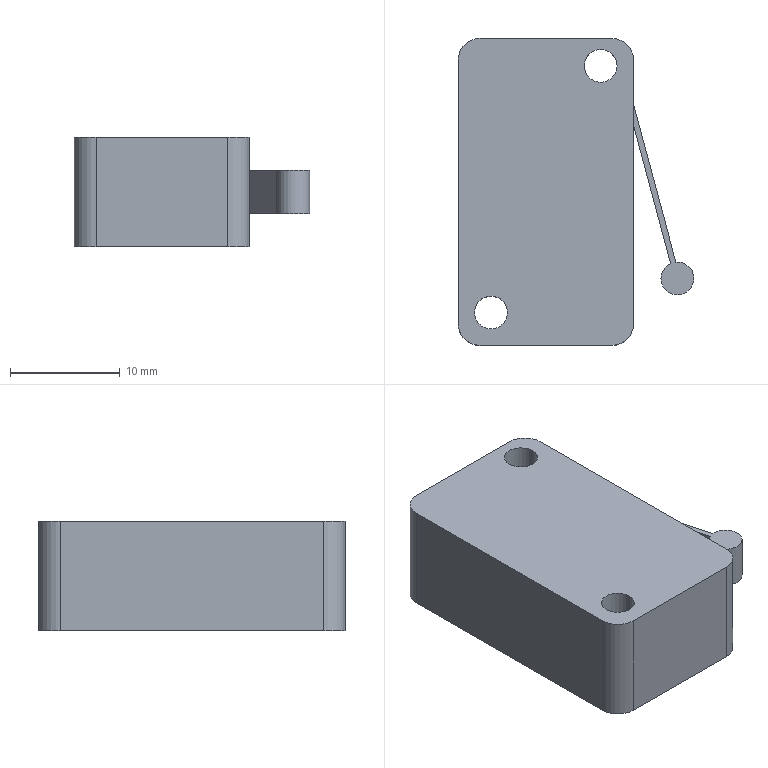Component | SolidWorks | MicroSwitch-1 | 2 solids | 22 faces | box 21.5 x 28 x 10 mm | volume 4360 mm3 | cylinder 11 | plane 11 | commonest cylinder face diameters 3 x7 4 x4
build123d program:
from build123d import *

# Parameters (mm, degrees)
SKETCH1_W      = 28
SKETCH1_H      = 16
EXTRUDE1_DEPTH = 5
SKETCH2_R      = 1.5
EXTRUDE2_DEPTH = 34.764
EXTRUDE3_DEPTH = 2
FILLET1_R      = 2


with BuildPart() as part:
    # Sketch1 → Extrude1 (new, symmetric)
    with BuildSketch(Plane(origin=(0, 0, 0), x_dir=(1, 0, 0), z_dir=(0, 1, 0))):
        with Locations((14, 8)):
            Rectangle(SKETCH1_W, SKETCH1_H)
    extrude(amount=EXTRUDE1_DEPTH, both=True)

    # Sketch2 → Extrude2 (cut, through all)
    with BuildSketch(Plane(origin=(0, 5, 0), x_dir=(1, 0, 0), z_dir=(0, 1, 0))):
        with Locations(Location((25.5, 13, 0), (0, 0, 270))):
            Circle(SKETCH2_R)
        with Locations(Location((3, 3, 0), (0, 0, 270))):
            Circle(SKETCH2_R)
    extrude(amount=-EXTRUDE2_DEPTH, mode=Mode.SUBTRACT)

    # Fillet1
    fillet1_edges = [part.edges().sort_by_distance(p)[0] for p in [
        (0, 0, -16),
        (28, 0, -16),
        (28, 0, 0),
        (0, 0, 0),
    ]]
    fillet(fillet1_edges, radius=FILLET1_R)


with BuildPart() as body_2:
    # Sketch3 → Extrude3 (new, symmetric)
    with BuildSketch(Plane(origin=(0, 0, 0), x_dir=(1, 0, 0), z_dir=(0, 1, 0))):
        with BuildLine():
            Line((7.599, 19.859), (22, 16))
            Line((22, 16), (20.068, 16))
            Line((20.068, 16), (7.47, 19.376))
            ThreePointArc((7.47, 19.376), (4.657, 20.388), (7.599, 19.859))
        make_face()
    extrude(amount=EXTRUDE3_DEPTH, both=True)


solid = Compound([part.part, body_2.part])

# Placed as in the assembly
solid = solid.moved(Location((-20.734, 63.799, 41), (-90, -90, 0)))
STEP:
#1=COLOUR_RGB('',0.7922,0.8196,0.9333);
#2=FILL_AREA_STYLE_COLOUR('',#1);
#3=FILL_AREA_STYLE('',(#2));
#4=SURFACE_STYLE_FILL_AREA(#3);
#5=SURFACE_SIDE_STYLE('',(#4));
#6=SURFACE_STYLE_USAGE(.BOTH.,#5);
#7=PRESENTATION_STYLE_ASSIGNMENT((#6));
#8=CARTESIAN_POINT('',(-0.6391,2.63,1.811));
#9=VERTEX_POINT('',#8);
#10=CARTESIAN_POINT('',(-0.7572,2.63,1.811));
#11=VERTEX_POINT('',#10);
#12=CARTESIAN_POINT('',(-0.6982,2.63,1.811));
#13=DIRECTION('',(-0.,0.,-1.));
#14=DIRECTION('',(-1.,0.,0.));
#15=AXIS2_PLACEMENT_3D('',#12,#13,#14);
#16=CIRCLE('',#15,0.05906);
#17=EDGE_CURVE('',#9,#11,#16,.T.);
#18=ORIENTED_EDGE('',*,*,#17,.F.);
#19=CARTESIAN_POINT('',(-0.6391,2.63,1.417));
#20=VERTEX_POINT('',#19);
#21=CARTESIAN_POINT('',(-0.6391,2.63,1.811));
#22=DIRECTION('',(-0.,0.,-1.));
#23=VECTOR('',#22,39.37);
#24=LINE('',#21,#23);
#25=EDGE_CURVE('',#9,#20,#24,.T.);
#26=ORIENTED_EDGE('',*,*,#25,.T.);
#27=CARTESIAN_POINT('',(-0.7572,2.63,1.417));
#28=VERTEX_POINT('',#27);
#29=CARTESIAN_POINT('',(-0.6982,2.63,1.417));
#30=DIRECTION('',(-0.,0.,-1.));
#31=DIRECTION('',(-1.,0.,0.));
#32=AXIS2_PLACEMENT_3D('',#29,#30,#31);
#33=CIRCLE('',#32,0.05906);
#34=EDGE_CURVE('',#20,#28,#33,.T.);
#35=ORIENTED_EDGE('',*,*,#34,.T.);
#36=CARTESIAN_POINT('',(-0.7572,2.63,1.811));
#37=DIRECTION('',(-0.,0.,-1.));
#38=VECTOR('',#37,39.37);
#39=LINE('',#36,#38);
#40=EDGE_CURVE('',#11,#28,#39,.T.);
#41=ORIENTED_EDGE('',*,*,#40,.F.);
#42=EDGE_LOOP('',(#18,#26,#35,#41));
#43=FACE_OUTER_BOUND('',#42,.T.);
#44=CARTESIAN_POINT('',(-0.6982,2.63,1.811));
#45=DIRECTION('',(-0.,0.,-1.));
#46=DIRECTION('',(-1.,0.,0.));
#47=AXIS2_PLACEMENT_3D('',#44,#45,#46);
#48=CYLINDRICAL_SURFACE('',#47,0.05906);
#49=ADVANCED_FACE('',(#43),#48,.F.);
#50=CARTESIAN_POINT('',(-0.2454,3.516,1.811));
#51=VERTEX_POINT('',#50);
#52=CARTESIAN_POINT('',(-0.3635,3.516,1.811));
#53=VERTEX_POINT('',#52);
#54=CARTESIAN_POINT('',(-0.3045,3.516,1.811));
#55=DIRECTION('',(-0.,0.,-1.));
#56=DIRECTION('',(-1.,0.,0.));
#57=AXIS2_PLACEMENT_3D('',#54,#55,#56);
#58=CIRCLE('',#57,0.05906);
#59=EDGE_CURVE('',#51,#53,#58,.T.);
#60=ORIENTED_EDGE('',*,*,#59,.F.);
#61=CARTESIAN_POINT('',(-0.2454,3.516,1.417));
#62=VERTEX_POINT('',#61);
#63=CARTESIAN_POINT('',(-0.2454,3.516,1.811));
#64=DIRECTION('',(-0.,0.,-1.));
#65=VECTOR('',#64,39.37);
#66=LINE('',#63,#65);
#67=EDGE_CURVE('',#51,#62,#66,.T.);
#68=ORIENTED_EDGE('',*,*,#67,.T.);
#69=CARTESIAN_POINT('',(-0.3635,3.516,1.417));
#70=VERTEX_POINT('',#69);
#71=CARTESIAN_POINT('',(-0.3045,3.516,1.417));
#72=DIRECTION('',(-0.,0.,-1.));
#73=DIRECTION('',(-1.,0.,0.));
#74=AXIS2_PLACEMENT_3D('',#71,#72,#73);
#75=CIRCLE('',#74,0.05906);
#76=EDGE_CURVE('',#62,#70,#75,.T.);
#77=ORIENTED_EDGE('',*,*,#76,.T.);
#78=CARTESIAN_POINT('',(-0.3635,3.516,1.811));
#79=DIRECTION('',(-0.,0.,-1.));
#80=VECTOR('',#79,39.37);
#81=LINE('',#78,#80);
#82=EDGE_CURVE('',#53,#70,#81,.T.);
#83=ORIENTED_EDGE('',*,*,#82,.F.);
#84=EDGE_LOOP('',(#60,#68,#77,#83));
#85=FACE_OUTER_BOUND('',#84,.T.);
#86=CARTESIAN_POINT('',(-0.3045,3.516,1.811));
#87=DIRECTION('',(-0.,0.,-1.));
#88=DIRECTION('',(-1.,0.,0.));
#89=AXIS2_PLACEMENT_3D('',#86,#87,#88);
#90=CYLINDRICAL_SURFACE('',#89,0.05906);
#91=ADVANCED_FACE('',(#85),#90,.F.);
#92=CARTESIAN_POINT('',(-0.2651,2.512,1.811));
#93=VERTEX_POINT('',#92);
#94=CARTESIAN_POINT('',(-0.7375,2.512,1.811));
#95=VERTEX_POINT('',#94);
#96=CARTESIAN_POINT('',(-0.8163,2.512,1.811));
#97=DIRECTION('',(-1.,-0.,0.));
#98=VECTOR('',#97,39.37);
#99=LINE('',#96,#98);
#100=EDGE_CURVE('',#93,#95,#99,.T.);
#101=ORIENTED_EDGE('',*,*,#100,.T.);
#102=CARTESIAN_POINT('',(-0.7375,2.512,1.417));
#103=VERTEX_POINT('',#102);
#104=CARTESIAN_POINT('',(-0.7375,2.512,1.417));
#105=DIRECTION('',(-0.,0.,-1.));
#106=VECTOR('',#105,39.37);
#107=LINE('',#104,#106);
#108=EDGE_CURVE('',#95,#103,#107,.T.);
#109=ORIENTED_EDGE('',*,*,#108,.T.);
#110=CARTESIAN_POINT('',(-0.2651,2.512,1.417));
#111=VERTEX_POINT('',#110);
#112=CARTESIAN_POINT('',(-0.8163,2.512,1.417));
#113=DIRECTION('',(-1.,-0.,0.));
#114=VECTOR('',#113,39.37);
#115=LINE('',#112,#114);
#116=EDGE_CURVE('',#111,#103,#115,.T.);
#117=ORIENTED_EDGE('',*,*,#116,.F.);
#118=CARTESIAN_POINT('',(-0.2651,2.512,1.417));
#119=DIRECTION('',(0.,-0.,1.));
#120=VECTOR('',#119,39.37);
#121=LINE('',#118,#120);
#122=EDGE_CURVE('',#111,#93,#121,.T.);
#123=ORIENTED_EDGE('',*,*,#122,.T.);
#124=EDGE_LOOP('',(#101,#109,#117,#123));
#125=FACE_OUTER_BOUND('',#124,.T.);
#126=CARTESIAN_POINT('',(-0.8163,2.512,1.417));
#127=DIRECTION('',(-0.,1.,0.));
#128=DIRECTION('',(1.,0.,-0.));
#129=AXIS2_PLACEMENT_3D('',#126,#127,#128);
#130=PLANE('',#129);
#131=ADVANCED_FACE('',(#125),#130,.F.);
#132=CARTESIAN_POINT('',(-0.8163,2.591,1.417));
#133=VERTEX_POINT('',#132);
#134=CARTESIAN_POINT('',(-0.8163,3.535,1.417));
#135=VERTEX_POINT('',#134);
#136=CARTESIAN_POINT('',(-0.8163,2.512,1.417));
#137=DIRECTION('',(-0.,1.,0.));
#138=VECTOR('',#137,39.37);
#139=LINE('',#136,#138);
#140=EDGE_CURVE('',#133,#135,#139,.T.);
#141=ORIENTED_EDGE('',*,*,#140,.F.);
#142=CARTESIAN_POINT('',(-0.8163,2.591,1.811));
#143=VERTEX_POINT('',#142);
#144=CARTESIAN_POINT('',(-0.8163,2.591,1.417));
#145=DIRECTION('',(0.,-0.,1.));
#146=VECTOR('',#145,39.37);
#147=LINE('',#144,#146);
#148=EDGE_CURVE('',#133,#143,#147,.T.);
#149=ORIENTED_EDGE('',*,*,#148,.T.);
#150=CARTESIAN_POINT('',(-0.8163,3.535,1.811));
#151=VERTEX_POINT('',#150);
#152=CARTESIAN_POINT('',(-0.8163,2.512,1.811));
#153=DIRECTION('',(-0.,1.,0.));
#154=VECTOR('',#153,39.37);
#155=LINE('',#152,#154);
#156=EDGE_CURVE('',#143,#151,#155,.T.);
#157=ORIENTED_EDGE('',*,*,#156,.T.);
#158=CARTESIAN_POINT('',(-0.8163,3.535,1.417));
#159=DIRECTION('',(-0.,0.,-1.));
#160=VECTOR('',#159,39.37);
#161=LINE('',#158,#160);
#162=EDGE_CURVE('',#151,#135,#161,.T.);
#163=ORIENTED_EDGE('',*,*,#162,.T.);
#164=EDGE_LOOP('',(#141,#149,#157,#163));
#165=FACE_OUTER_BOUND('',#164,.T.);
#166=CARTESIAN_POINT('',(-0.8163,2.512,1.417));
#167=DIRECTION('',(1.,0.,-0.));
#168=DIRECTION('',(0.,-1.,-0.));
#169=AXIS2_PLACEMENT_3D('',#166,#167,#168);
#170=PLANE('',#169);
#171=ADVANCED_FACE('',(#165),#170,.F.);
#172=CARTESIAN_POINT('',(-0.7375,3.614,1.417));
#173=VERTEX_POINT('',#172);
#174=CARTESIAN_POINT('',(-0.2651,3.614,1.417));
#175=VERTEX_POINT('',#174);
#176=CARTESIAN_POINT('',(-0.8163,3.614,1.417));
#177=DIRECTION('',(1.,-0.,-0.));
#178=VECTOR('',#177,39.37);
#179=LINE('',#176,#178);
#180=EDGE_CURVE('',#173,#175,#179,.T.);
#181=ORIENTED_EDGE('',*,*,#180,.F.);
#182=CARTESIAN_POINT('',(-0.7375,3.614,1.811));
#183=VERTEX_POINT('',#182);
#184=CARTESIAN_POINT('',(-0.7375,3.614,1.417));
#185=DIRECTION('',(0.,-0.,1.));
#186=VECTOR('',#185,39.37);
#187=LINE('',#184,#186);
#188=EDGE_CURVE('',#173,#183,#187,.T.);
#189=ORIENTED_EDGE('',*,*,#188,.T.);
#190=CARTESIAN_POINT('',(-0.2651,3.614,1.811));
#191=VERTEX_POINT('',#190);
#192=CARTESIAN_POINT('',(-0.8163,3.614,1.811));
#193=DIRECTION('',(1.,-0.,-0.));
#194=VECTOR('',#193,39.37);
#195=LINE('',#192,#194);
#196=EDGE_CURVE('',#183,#191,#195,.T.);
#197=ORIENTED_EDGE('',*,*,#196,.T.);
#198=CARTESIAN_POINT('',(-0.2651,3.614,1.417));
#199=DIRECTION('',(-0.,0.,-1.));
#200=VECTOR('',#199,39.37);
#201=LINE('',#198,#200);
#202=EDGE_CURVE('',#191,#175,#201,.T.);
#203=ORIENTED_EDGE('',*,*,#202,.T.);
#204=EDGE_LOOP('',(#181,#189,#197,#203));
#205=FACE_OUTER_BOUND('',#204,.T.);
#206=CARTESIAN_POINT('',(-0.8163,3.614,1.417));
#207=DIRECTION('',(-0.,-1.,-0.));
#208=DIRECTION('',(-1.,0.,0.));
#209=AXIS2_PLACEMENT_3D('',#206,#207,#208);
#210=PLANE('',#209);
#211=ADVANCED_FACE('',(#205),#210,.F.);
#212=CARTESIAN_POINT('',(-0.1864,3.535,1.417));
#213=VERTEX_POINT('',#212);
#214=CARTESIAN_POINT('',(-0.1864,2.591,1.417));
#215=VERTEX_POINT('',#214);
#216=CARTESIAN_POINT('',(-0.1864,2.512,1.417));
#217=DIRECTION('',(0.,-1.,-0.));
#218=VECTOR('',#217,39.37);
#219=LINE('',#216,#218);
#220=EDGE_CURVE('',#213,#215,#219,.T.);
#221=ORIENTED_EDGE('',*,*,#220,.F.);
#222=CARTESIAN_POINT('',(-0.1864,3.535,1.811));
#223=VERTEX_POINT('',#222);
#224=CARTESIAN_POINT('',(-0.1864,3.535,1.417));
#225=DIRECTION('',(0.,-0.,1.));
#226=VECTOR('',#225,39.37);
#227=LINE('',#224,#226);
#228=EDGE_CURVE('',#213,#223,#227,.T.);
#229=ORIENTED_EDGE('',*,*,#228,.T.);
#230=CARTESIAN_POINT('',(-0.1864,2.591,1.811));
#231=VERTEX_POINT('',#230);
#232=CARTESIAN_POINT('',(-0.1864,2.512,1.811));
#233=DIRECTION('',(0.,-1.,-0.));
#234=VECTOR('',#233,39.37);
#235=LINE('',#232,#234);
#236=EDGE_CURVE('',#223,#231,#235,.T.);
#237=ORIENTED_EDGE('',*,*,#236,.T.);
#238=CARTESIAN_POINT('',(-0.1864,2.591,1.417));
#239=DIRECTION('',(-0.,0.,-1.));
#240=VECTOR('',#239,39.37);
#241=LINE('',#238,#240);
#242=EDGE_CURVE('',#231,#215,#241,.T.);
#243=ORIENTED_EDGE('',*,*,#242,.T.);
#244=EDGE_LOOP('',(#221,#229,#237,#243));
#245=FACE_OUTER_BOUND('',#244,.T.);
#246=CARTESIAN_POINT('',(-0.1864,2.512,1.417));
#247=DIRECTION('',(-1.,-0.,0.));
#248=DIRECTION('',(-0.,1.,0.));
#249=AXIS2_PLACEMENT_3D('',#246,#247,#248);
#250=PLANE('',#249);
#251=ADVANCED_FACE('',(#245),#250,.F.);
#252=CARTESIAN_POINT('',(-0.6982,2.63,1.417));
#253=DIRECTION('',(-0.,0.,-1.));
#254=DIRECTION('',(-1.,0.,0.));
#255=AXIS2_PLACEMENT_3D('',#252,#253,#254);
#256=CIRCLE('',#255,0.05906);
#257=EDGE_CURVE('',#28,#20,#256,.T.);
#258=ORIENTED_EDGE('',*,*,#257,.F.);
#259=ORIENTED_EDGE('',*,*,#34,.F.);
#260=EDGE_LOOP('',(#258,#259));
#261=FACE_BOUND('',#260,.T.);
#262=CARTESIAN_POINT('',(-0.3045,3.516,1.417));
#263=DIRECTION('',(-0.,0.,-1.));
#264=DIRECTION('',(-1.,0.,0.));
#265=AXIS2_PLACEMENT_3D('',#262,#263,#264);
#266=CIRCLE('',#265,0.05906);
#267=EDGE_CURVE('',#70,#62,#266,.T.);
#268=ORIENTED_EDGE('',*,*,#267,.F.);
#269=ORIENTED_EDGE('',*,*,#76,.F.);
#270=EDGE_LOOP('',(#268,#269));
#271=FACE_BOUND('',#270,.T.);
#272=ORIENTED_EDGE('',*,*,#116,.T.);
#273=CARTESIAN_POINT('',(-0.7375,2.591,1.417));
#274=DIRECTION('',(-0.,0.,-1.));
#275=DIRECTION('',(1.,0.,0.));
#276=AXIS2_PLACEMENT_3D('',#273,#274,#275);
#277=CIRCLE('',#276,0.07874);
#278=EDGE_CURVE('',#103,#133,#277,.T.);
#279=ORIENTED_EDGE('',*,*,#278,.T.);
#280=ORIENTED_EDGE('',*,*,#140,.T.);
#281=CARTESIAN_POINT('',(-0.7375,3.535,1.417));
#282=DIRECTION('',(-0.,0.,-1.));
#283=DIRECTION('',(1.,0.,0.));
#284=AXIS2_PLACEMENT_3D('',#281,#282,#283);
#285=CIRCLE('',#284,0.07874);
#286=EDGE_CURVE('',#135,#173,#285,.T.);
#287=ORIENTED_EDGE('',*,*,#286,.T.);
#288=ORIENTED_EDGE('',*,*,#180,.T.);
#289=CARTESIAN_POINT('',(-0.2651,3.535,1.417));
#290=DIRECTION('',(-0.,0.,-1.));
#291=DIRECTION('',(1.,0.,0.));
#292=AXIS2_PLACEMENT_3D('',#289,#290,#291);
#293=CIRCLE('',#292,0.07874);
#294=EDGE_CURVE('',#175,#213,#293,.T.);
#295=ORIENTED_EDGE('',*,*,#294,.T.);
#296=ORIENTED_EDGE('',*,*,#220,.T.);
#297=CARTESIAN_POINT('',(-0.2651,2.591,1.417));
#298=DIRECTION('',(-0.,0.,-1.));
#299=DIRECTION('',(1.,0.,0.));
#300=AXIS2_PLACEMENT_3D('',#297,#298,#299);
#301=CIRCLE('',#300,0.07874);
#302=EDGE_CURVE('',#215,#111,#301,.T.);
#303=ORIENTED_EDGE('',*,*,#302,.T.);
#304=EDGE_LOOP('',(#272,#279,#280,#287,#288,#295,#296,#303));
#305=FACE_OUTER_BOUND('',#304,.T.);
#306=CARTESIAN_POINT('',(-0.1864,2.512,1.417));
#307=DIRECTION('',(0.,-0.,1.));
#308=DIRECTION('',(1.,0.,-0.));
#309=AXIS2_PLACEMENT_3D('',#306,#307,#308);
#310=PLANE('',#309);
#311=ADVANCED_FACE('',(#261,#271,#305),#310,.F.);
#312=CARTESIAN_POINT('',(-0.6982,2.63,1.811));
#313=DIRECTION('',(-0.,0.,-1.));
#314=DIRECTION('',(-1.,0.,0.));
#315=AXIS2_PLACEMENT_3D('',#312,#313,#314);
#316=CIRCLE('',#315,0.05906);
#317=EDGE_CURVE('',#11,#9,#316,.T.);
#318=ORIENTED_EDGE('',*,*,#317,.T.);
#319=ORIENTED_EDGE('',*,*,#17,.T.);
#320=EDGE_LOOP('',(#318,#319));
#321=FACE_BOUND('',#320,.T.);
#322=CARTESIAN_POINT('',(-0.3045,3.516,1.811));
#323=DIRECTION('',(-0.,0.,-1.));
#324=DIRECTION('',(-1.,0.,0.));
#325=AXIS2_PLACEMENT_3D('',#322,#323,#324);
#326=CIRCLE('',#325,0.05906);
#327=EDGE_CURVE('',#53,#51,#326,.T.);
#328=ORIENTED_EDGE('',*,*,#327,.T.);
#329=ORIENTED_EDGE('',*,*,#59,.T.);
#330=EDGE_LOOP('',(#328,#329));
#331=FACE_BOUND('',#330,.T.);
#332=ORIENTED_EDGE('',*,*,#156,.F.);
#333=CARTESIAN_POINT('',(-0.7375,2.591,1.811));
#334=DIRECTION('',(0.,-0.,1.));
#335=DIRECTION('',(1.,0.,0.));
#336=AXIS2_PLACEMENT_3D('',#333,#334,#335);
#337=CIRCLE('',#336,0.07874);
#338=EDGE_CURVE('',#143,#95,#337,.T.);
#339=ORIENTED_EDGE('',*,*,#338,.T.);
#340=ORIENTED_EDGE('',*,*,#100,.F.);
#341=CARTESIAN_POINT('',(-0.2651,2.591,1.811));
#342=DIRECTION('',(0.,-0.,1.));
#343=DIRECTION('',(1.,0.,0.));
#344=AXIS2_PLACEMENT_3D('',#341,#342,#343);
#345=CIRCLE('',#344,0.07874);
#346=EDGE_CURVE('',#93,#231,#345,.T.);
#347=ORIENTED_EDGE('',*,*,#346,.T.);
#348=ORIENTED_EDGE('',*,*,#236,.F.);
#349=CARTESIAN_POINT('',(-0.2651,3.535,1.811));
#350=DIRECTION('',(0.,-0.,1.));
#351=DIRECTION('',(1.,0.,0.));
#352=AXIS2_PLACEMENT_3D('',#349,#350,#351);
#353=CIRCLE('',#352,0.07874);
#354=EDGE_CURVE('',#223,#191,#353,.T.);
#355=ORIENTED_EDGE('',*,*,#354,.T.);
#356=ORIENTED_EDGE('',*,*,#196,.F.);
#357=CARTESIAN_POINT('',(-0.7375,3.535,1.811));
#358=DIRECTION('',(0.,-0.,1.));
#359=DIRECTION('',(1.,0.,0.));
#360=AXIS2_PLACEMENT_3D('',#357,#358,#359);
#361=CIRCLE('',#360,0.07874);
#362=EDGE_CURVE('',#183,#151,#361,.T.);
#363=ORIENTED_EDGE('',*,*,#362,.T.);
#364=EDGE_LOOP('',(#332,#339,#340,#347,#348,#355,#356,#363));
#365=FACE_OUTER_BOUND('',#364,.T.);
#366=CARTESIAN_POINT('',(-0.1864,2.512,1.811));
#367=DIRECTION('',(0.,-0.,1.));
#368=DIRECTION('',(1.,0.,-0.));
#369=AXIS2_PLACEMENT_3D('',#366,#367,#368);
#370=PLANE('',#369);
#371=ADVANCED_FACE('',(#321,#331,#365),#370,.T.);
#372=ORIENTED_EDGE('',*,*,#67,.F.);
#373=ORIENTED_EDGE('',*,*,#327,.F.);
#374=ORIENTED_EDGE('',*,*,#82,.T.);
#375=ORIENTED_EDGE('',*,*,#267,.T.);
#376=EDGE_LOOP('',(#372,#373,#374,#375));
#377=FACE_OUTER_BOUND('',#376,.T.);
#378=CARTESIAN_POINT('',(-0.3045,3.516,1.811));
#379=DIRECTION('',(-0.,0.,-1.));
#380=DIRECTION('',(-1.,0.,0.));
#381=AXIS2_PLACEMENT_3D('',#378,#379,#380);
#382=CYLINDRICAL_SURFACE('',#381,0.05906);
#383=ADVANCED_FACE('',(#377),#382,.F.);
#384=ORIENTED_EDGE('',*,*,#25,.F.);
#385=ORIENTED_EDGE('',*,*,#317,.F.);
#386=ORIENTED_EDGE('',*,*,#40,.T.);
#387=ORIENTED_EDGE('',*,*,#257,.T.);
#388=EDGE_LOOP('',(#384,#385,#386,#387));
#389=FACE_OUTER_BOUND('',#388,.T.);
#390=CARTESIAN_POINT('',(-0.6982,2.63,1.811));
#391=DIRECTION('',(-0.,0.,-1.));
#392=DIRECTION('',(-1.,0.,0.));
#393=AXIS2_PLACEMENT_3D('',#390,#391,#392);
#394=CYLINDRICAL_SURFACE('',#393,0.05906);
#395=ADVANCED_FACE('',(#389),#394,.F.);
#396=ORIENTED_EDGE('',*,*,#278,.F.);
#397=ORIENTED_EDGE('',*,*,#108,.F.);
#398=ORIENTED_EDGE('',*,*,#338,.F.);
#399=ORIENTED_EDGE('',*,*,#148,.F.);
#400=EDGE_LOOP('',(#396,#397,#398,#399));
#401=FACE_OUTER_BOUND('',#400,.T.);
#402=CARTESIAN_POINT('',(-0.7375,2.591,1.417));
#403=DIRECTION('',(0.,-0.,1.));
#404=DIRECTION('',(1.,0.,0.));
#405=AXIS2_PLACEMENT_3D('',#402,#403,#404);
#406=CYLINDRICAL_SURFACE('',#405,0.07874);
#407=ADVANCED_FACE('',(#401),#406,.T.);
#408=ORIENTED_EDGE('',*,*,#286,.F.);
#409=ORIENTED_EDGE('',*,*,#162,.F.);
#410=ORIENTED_EDGE('',*,*,#362,.F.);
#411=ORIENTED_EDGE('',*,*,#188,.F.);
#412=EDGE_LOOP('',(#408,#409,#410,#411));
#413=FACE_OUTER_BOUND('',#412,.T.);
#414=CARTESIAN_POINT('',(-0.7375,3.535,1.417));
#415=DIRECTION('',(0.,-0.,1.));
#416=DIRECTION('',(1.,0.,0.));
#417=AXIS2_PLACEMENT_3D('',#414,#415,#416);
#418=CYLINDRICAL_SURFACE('',#417,0.07874);
#419=ADVANCED_FACE('',(#413),#418,.T.);
#420=ORIENTED_EDGE('',*,*,#294,.F.);
#421=ORIENTED_EDGE('',*,*,#202,.F.);
#422=ORIENTED_EDGE('',*,*,#354,.F.);
#423=ORIENTED_EDGE('',*,*,#228,.F.);
#424=EDGE_LOOP('',(#420,#421,#422,#423));
#425=FACE_OUTER_BOUND('',#424,.T.);
#426=CARTESIAN_POINT('',(-0.2651,3.535,1.417));
#427=DIRECTION('',(0.,-0.,1.));
#428=DIRECTION('',(1.,0.,0.));
#429=AXIS2_PLACEMENT_3D('',#426,#427,#428);
#430=CYLINDRICAL_SURFACE('',#429,0.07874);
#431=ADVANCED_FACE('',(#425),#430,.T.);
#432=ORIENTED_EDGE('',*,*,#302,.F.);
#433=ORIENTED_EDGE('',*,*,#242,.F.);
#434=ORIENTED_EDGE('',*,*,#346,.F.);
#435=ORIENTED_EDGE('',*,*,#122,.F.);
#436=EDGE_LOOP('',(#432,#433,#434,#435));
#437=FACE_OUTER_BOUND('',#436,.T.);
#438=CARTESIAN_POINT('',(-0.2651,2.591,1.417));
#439=DIRECTION('',(0.,-0.,1.));
#440=DIRECTION('',(1.,0.,0.));
#441=AXIS2_PLACEMENT_3D('',#438,#439,#440);
#442=CYLINDRICAL_SURFACE('',#441,0.07874);
#443=ADVANCED_FACE('',(#437),#442,.T.);
#444=CLOSED_SHELL('',(#49,#91,#131,#171,#211,#251,#311,#371,#383,#395,#407,#419,#431,#443));
#445=MANIFOLD_SOLID_BREP('',#444);
#446=STYLED_ITEM('',(#7),#445);
#447=PRESENTATION_LAYER_ASSIGNMENT('','',(#446));
#448=COLOUR_RGB('',0.7922,0.8196,0.9333);
#449=FILL_AREA_STYLE_COLOUR('',#448);
#450=FILL_AREA_STYLE('',(#449));
#451=SURFACE_STYLE_FILL_AREA(#450);
#452=SURFACE_SIDE_STYLE('',(#451));
#453=SURFACE_STYLE_USAGE(.BOTH.,#452);
#454=PRESENTATION_STYLE_ASSIGNMENT((#453));
#455=CARTESIAN_POINT('',(-0.03445,2.811,1.693));
#456=VERTEX_POINT('',#455);
#457=CARTESIAN_POINT('',(0.03017,2.752,1.693));
#458=VERTEX_POINT('',#457);
#459=CARTESIAN_POINT('',(-0.02889,2.752,1.693));
#460=DIRECTION('',(-0.,0.,-1.));
#461=DIRECTION('',(-1.,0.,0.));
#462=AXIS2_PLACEMENT_3D('',#459,#460,#461);
#463=CIRCLE('',#462,0.05906);
#464=EDGE_CURVE('',#456,#458,#463,.T.);
#465=ORIENTED_EDGE('',*,*,#464,.T.);
#466=CARTESIAN_POINT('',(0.03017,2.752,1.535));
#467=VERTEX_POINT('',#466);
#468=CARTESIAN_POINT('',(0.03017,2.752,1.693));
#469=DIRECTION('',(-0.,0.,-1.));
#470=VECTOR('',#469,39.37);
#471=LINE('',#468,#470);
#472=EDGE_CURVE('',#458,#467,#471,.T.);
#473=ORIENTED_EDGE('',*,*,#472,.T.);
#474=CARTESIAN_POINT('',(-0.03445,2.811,1.535));
#475=VERTEX_POINT('',#474);
#476=CARTESIAN_POINT('',(-0.02889,2.752,1.535));
#477=DIRECTION('',(-0.,0.,-1.));
#478=DIRECTION('',(-1.,0.,0.));
#479=AXIS2_PLACEMENT_3D('',#476,#477,#478);
#480=CIRCLE('',#479,0.05906);
#481=EDGE_CURVE('',#475,#467,#480,.T.);
#482=ORIENTED_EDGE('',*,*,#481,.F.);
#483=CARTESIAN_POINT('',(-0.03445,2.811,1.693));
#484=DIRECTION('',(-0.,0.,-1.));
#485=VECTOR('',#484,39.37);
#486=LINE('',#483,#485);
#487=EDGE_CURVE('',#456,#475,#486,.T.);
#488=ORIENTED_EDGE('',*,*,#487,.F.);
#489=EDGE_LOOP('',(#465,#473,#482,#488));
#490=FACE_OUTER_BOUND('',#489,.T.);
#491=CARTESIAN_POINT('',(-0.02889,2.752,1.693));
#492=DIRECTION('',(-0.,0.,-1.));
#493=DIRECTION('',(-1.,0.,0.));
#494=AXIS2_PLACEMENT_3D('',#491,#492,#493);
#495=CYLINDRICAL_SURFACE('',#494,0.05906);
#496=ADVANCED_FACE('',(#490),#495,.T.);
#497=ORIENTED_EDGE('',*,*,#472,.F.);
#498=CARTESIAN_POINT('',(-0.08794,2.752,1.693));
#499=VERTEX_POINT('',#498);
#500=CARTESIAN_POINT('',(-0.02889,2.752,1.693));
#501=DIRECTION('',(-0.,0.,-1.));
#502=DIRECTION('',(-1.,0.,0.));
#503=AXIS2_PLACEMENT_3D('',#500,#501,#502);
#504=CIRCLE('',#503,0.05906);
#505=EDGE_CURVE('',#458,#499,#504,.T.);
#506=ORIENTED_EDGE('',*,*,#505,.T.);
#507=CARTESIAN_POINT('',(-0.08794,2.752,1.535));
#508=VERTEX_POINT('',#507);
#509=CARTESIAN_POINT('',(-0.08794,2.752,1.693));
#510=DIRECTION('',(-0.,0.,-1.));
#511=VECTOR('',#510,39.37);
#512=LINE('',#509,#511);
#513=EDGE_CURVE('',#499,#508,#512,.T.);
#514=ORIENTED_EDGE('',*,*,#513,.T.);
#515=CARTESIAN_POINT('',(-0.02889,2.752,1.535));
#516=DIRECTION('',(-0.,0.,-1.));
#517=DIRECTION('',(-1.,0.,0.));
#518=AXIS2_PLACEMENT_3D('',#515,#516,#517);
#519=CIRCLE('',#518,0.05906);
#520=EDGE_CURVE('',#467,#508,#519,.T.);
#521=ORIENTED_EDGE('',*,*,#520,.F.);
#522=EDGE_LOOP('',(#497,#506,#514,#521));
#523=FACE_OUTER_BOUND('',#522,.T.);
#524=CARTESIAN_POINT('',(-0.02889,2.752,1.693));
#525=DIRECTION('',(-0.,0.,-1.));
#526=DIRECTION('',(-1.,0.,0.));
#527=AXIS2_PLACEMENT_3D('',#524,#525,#526);
#528=CYLINDRICAL_SURFACE('',#527,0.05906);
#529=ADVANCED_FACE('',(#523),#528,.T.);
#530=ORIENTED_EDGE('',*,*,#513,.F.);
#531=CARTESIAN_POINT('',(-0.05346,2.806,1.693));
#532=VERTEX_POINT('',#531);
#533=CARTESIAN_POINT('',(-0.02889,2.752,1.693));
#534=DIRECTION('',(-0.,0.,-1.));
#535=DIRECTION('',(-1.,0.,0.));
#536=AXIS2_PLACEMENT_3D('',#533,#534,#535);
#537=CIRCLE('',#536,0.05906);
#538=EDGE_CURVE('',#499,#532,#537,.T.);
#539=ORIENTED_EDGE('',*,*,#538,.T.);
#540=CARTESIAN_POINT('',(-0.05346,2.806,1.535));
#541=VERTEX_POINT('',#540);
#542=CARTESIAN_POINT('',(-0.05346,2.806,1.693));
#543=DIRECTION('',(-0.,0.,-1.));
#544=VECTOR('',#543,39.37);
#545=LINE('',#542,#544);
#546=EDGE_CURVE('',#532,#541,#545,.T.);
#547=ORIENTED_EDGE('',*,*,#546,.T.);
#548=CARTESIAN_POINT('',(-0.02889,2.752,1.535));
#549=DIRECTION('',(-0.,0.,-1.));
#550=DIRECTION('',(-1.,0.,0.));
#551=AXIS2_PLACEMENT_3D('',#548,#549,#550);
#552=CIRCLE('',#551,0.05906);
#553=EDGE_CURVE('',#508,#541,#552,.T.);
#554=ORIENTED_EDGE('',*,*,#553,.F.);
#555=EDGE_LOOP('',(#530,#539,#547,#554));
#556=FACE_OUTER_BOUND('',#555,.T.);
#557=CARTESIAN_POINT('',(-0.02889,2.752,1.693));
#558=DIRECTION('',(-0.,0.,-1.));
#559=DIRECTION('',(-1.,0.,0.));
#560=AXIS2_PLACEMENT_3D('',#557,#558,#559);
#561=CYLINDRICAL_SURFACE('',#560,0.05906);
#562=ADVANCED_FACE('',(#556),#561,.T.);
#563=CARTESIAN_POINT('',(-0.1864,3.378,1.535));
#564=VERTEX_POINT('',#563);
#565=CARTESIAN_POINT('',(-0.03445,2.811,1.535));
#566=DIRECTION('',(0.2588,-0.9659,-0.));
#567=VECTOR('',#566,39.37);
#568=LINE('',#565,#567);
#569=EDGE_CURVE('',#564,#475,#568,.T.);
#570=ORIENTED_EDGE('',*,*,#569,.F.);
#571=CARTESIAN_POINT('',(-0.1864,3.378,1.693));
#572=VERTEX_POINT('',#571);
#573=CARTESIAN_POINT('',(-0.1864,3.378,1.693));
#574=DIRECTION('',(-0.,0.,-1.));
#575=VECTOR('',#574,39.37);
#576=LINE('',#573,#575);
#577=EDGE_CURVE('',#572,#564,#576,.T.);
#578=ORIENTED_EDGE('',*,*,#577,.F.);
#579=CARTESIAN_POINT('',(-0.03445,2.811,1.693));
#580=DIRECTION('',(0.2588,-0.9659,-0.));
#581=VECTOR('',#580,39.37);
#582=LINE('',#579,#581);
#583=EDGE_CURVE('',#572,#456,#582,.T.);
#584=ORIENTED_EDGE('',*,*,#583,.T.);
#585=ORIENTED_EDGE('',*,*,#487,.T.);
#586=EDGE_LOOP('',(#570,#578,#584,#585));
#587=FACE_OUTER_BOUND('',#586,.T.);
#588=CARTESIAN_POINT('',(-0.03445,2.811,1.693));
#589=DIRECTION('',(0.9659,0.2588,0.));
#590=DIRECTION('',(0.2588,-0.9659,-0.));
#591=AXIS2_PLACEMENT_3D('',#588,#589,#590);
#592=PLANE('',#591);
#593=ADVANCED_FACE('',(#587),#592,.T.);
#594=CARTESIAN_POINT('',(-0.1864,3.302,1.535));
#595=VERTEX_POINT('',#594);
#596=CARTESIAN_POINT('',(-0.1864,3.378,1.535));
#597=DIRECTION('',(-0.,1.,0.));
#598=VECTOR('',#597,39.37);
#599=LINE('',#596,#598);
#600=EDGE_CURVE('',#595,#564,#599,.T.);
#601=ORIENTED_EDGE('',*,*,#600,.F.);
#602=CARTESIAN_POINT('',(-0.1864,3.302,1.693));
#603=VERTEX_POINT('',#602);
#604=CARTESIAN_POINT('',(-0.1864,3.302,1.693));
#605=DIRECTION('',(-0.,0.,-1.));
#606=VECTOR('',#605,39.37);
#607=LINE('',#604,#606);
#608=EDGE_CURVE('',#603,#595,#607,.T.);
#609=ORIENTED_EDGE('',*,*,#608,.F.);
#610=CARTESIAN_POINT('',(-0.1864,3.378,1.693));
#611=DIRECTION('',(-0.,1.,0.));
#612=VECTOR('',#611,39.37);
#613=LINE('',#610,#612);
#614=EDGE_CURVE('',#603,#572,#613,.T.);
#615=ORIENTED_EDGE('',*,*,#614,.T.);
#616=ORIENTED_EDGE('',*,*,#577,.T.);
#617=EDGE_LOOP('',(#601,#609,#615,#616));
#618=FACE_OUTER_BOUND('',#617,.T.);
#619=CARTESIAN_POINT('',(-0.1864,3.378,1.693));
#620=DIRECTION('',(-1.,-0.,0.));
#621=DIRECTION('',(-0.,1.,0.));
#622=AXIS2_PLACEMENT_3D('',#619,#620,#621);
#623=PLANE('',#622);
#624=ADVANCED_FACE('',(#618),#623,.T.);
#625=CARTESIAN_POINT('',(-0.1864,3.302,1.535));
#626=DIRECTION('',(-0.2588,0.9659,0.));
#627=VECTOR('',#626,39.37);
#628=LINE('',#625,#627);
#629=EDGE_CURVE('',#541,#595,#628,.T.);
#630=ORIENTED_EDGE('',*,*,#629,.F.);
#631=ORIENTED_EDGE('',*,*,#546,.F.);
#632=CARTESIAN_POINT('',(-0.1864,3.302,1.693));
#633=DIRECTION('',(-0.2588,0.9659,0.));
#634=VECTOR('',#633,39.37);
#635=LINE('',#632,#634);
#636=EDGE_CURVE('',#532,#603,#635,.T.);
#637=ORIENTED_EDGE('',*,*,#636,.T.);
#638=ORIENTED_EDGE('',*,*,#608,.T.);
#639=EDGE_LOOP('',(#630,#631,#637,#638));
#640=FACE_OUTER_BOUND('',#639,.T.);
#641=CARTESIAN_POINT('',(-0.1864,3.302,1.693));
#642=DIRECTION('',(-0.9659,-0.2588,-0.));
#643=DIRECTION('',(-0.2588,0.9659,0.));
#644=AXIS2_PLACEMENT_3D('',#641,#642,#643);
#645=PLANE('',#644);
#646=ADVANCED_FACE('',(#640),#645,.T.);
#647=ORIENTED_EDGE('',*,*,#464,.F.);
#648=ORIENTED_EDGE('',*,*,#583,.F.);
#649=ORIENTED_EDGE('',*,*,#614,.F.);
#650=ORIENTED_EDGE('',*,*,#636,.F.);
#651=ORIENTED_EDGE('',*,*,#538,.F.);
#652=ORIENTED_EDGE('',*,*,#505,.F.);
#653=EDGE_LOOP('',(#647,#648,#649,#650,#651,#652));
#654=FACE_OUTER_BOUND('',#653,.T.);
#655=CARTESIAN_POINT('',(-0.02889,2.752,1.693));
#656=DIRECTION('',(-0.,0.,-1.));
#657=DIRECTION('',(-1.,-0.,0.));
#658=AXIS2_PLACEMENT_3D('',#655,#656,#657);
#659=PLANE('',#658);
#660=ADVANCED_FACE('',(#654),#659,.F.);
#661=ORIENTED_EDGE('',*,*,#481,.T.);
#662=ORIENTED_EDGE('',*,*,#520,.T.);
#663=ORIENTED_EDGE('',*,*,#553,.T.);
#664=ORIENTED_EDGE('',*,*,#629,.T.);
#665=ORIENTED_EDGE('',*,*,#600,.T.);
#666=ORIENTED_EDGE('',*,*,#569,.T.);
#667=EDGE_LOOP('',(#661,#662,#663,#664,#665,#666));
#668=FACE_OUTER_BOUND('',#667,.T.);
#669=CARTESIAN_POINT('',(-0.02889,2.752,1.535));
#670=DIRECTION('',(-0.,0.,-1.));
#671=DIRECTION('',(-1.,-0.,0.));
#672=AXIS2_PLACEMENT_3D('',#669,#670,#671);
#673=PLANE('',#672);
#674=ADVANCED_FACE('',(#668),#673,.T.);
#675=CLOSED_SHELL('',(#496,#529,#562,#593,#624,#646,#660,#674));
#676=MANIFOLD_SOLID_BREP('',#675);
#677=STYLED_ITEM('',(#454),#676);
#678=PRESENTATION_LAYER_ASSIGNMENT('','',(#677));
#679=(LENGTH_UNIT()NAMED_UNIT(*)SI_UNIT($,.METRE.));
#680=LENGTH_MEASURE_WITH_UNIT(LENGTH_MEASURE(0.0254),#679);
#681=DIMENSIONAL_EXPONENTS(1.,0.,0.,0.,0.,0.,0.);
#682=(CONVERSION_BASED_UNIT('',#680)LENGTH_UNIT()NAMED_UNIT(#681));
#683=UNCERTAINTY_MEASURE_WITH_UNIT(LENGTH_MEASURE(0.00001),#682,'','');
#684=(NAMED_UNIT(*)PLANE_ANGLE_UNIT()SI_UNIT($,.RADIAN.));
#685=(NAMED_UNIT(*)SI_UNIT($,.STERADIAN.)SOLID_ANGLE_UNIT());
#686=(GEOMETRIC_REPRESENTATION_CONTEXT(3)GLOBAL_UNCERTAINTY_ASSIGNED_CONTEXT((#683))GLOBAL_UNIT_ASSIGNED_CONTEXT((#682,#684,#685))REPRESENTATION_CONTEXT('',''));
#687=MECHANICAL_DESIGN_GEOMETRIC_PRESENTATION_REPRESENTATION('',(#446),#686);
#688=(LENGTH_UNIT()NAMED_UNIT(*)SI_UNIT($,.METRE.));
#689=LENGTH_MEASURE_WITH_UNIT(LENGTH_MEASURE(0.0254),#688);
#690=DIMENSIONAL_EXPONENTS(1.,0.,0.,0.,0.,0.,0.);
#691=(CONVERSION_BASED_UNIT('',#689)LENGTH_UNIT()NAMED_UNIT(#690));
#692=UNCERTAINTY_MEASURE_WITH_UNIT(LENGTH_MEASURE(0.00001),#691,'','');
#693=(NAMED_UNIT(*)PLANE_ANGLE_UNIT()SI_UNIT($,.RADIAN.));
#694=(NAMED_UNIT(*)SI_UNIT($,.STERADIAN.)SOLID_ANGLE_UNIT());
#695=(GEOMETRIC_REPRESENTATION_CONTEXT(3)GLOBAL_UNCERTAINTY_ASSIGNED_CONTEXT((#692))GLOBAL_UNIT_ASSIGNED_CONTEXT((#691,#693,#694))REPRESENTATION_CONTEXT('',''));
#696=MECHANICAL_DESIGN_GEOMETRIC_PRESENTATION_REPRESENTATION('',(#677),#695);
#697=CARTESIAN_POINT('',(0.,0.,0.));
#698=DIRECTION('',(0.,0.,1.));
#699=DIRECTION('',(1.,0.,0.));
#700=AXIS2_PLACEMENT_3D('',#697,#698,#699);
#701=(LENGTH_UNIT()NAMED_UNIT(*)SI_UNIT($,.METRE.));
#702=LENGTH_MEASURE_WITH_UNIT(LENGTH_MEASURE(0.0254),#701);
#703=DIMENSIONAL_EXPONENTS(1.,0.,0.,0.,0.,0.,0.);
#704=(CONVERSION_BASED_UNIT('',#702)LENGTH_UNIT()NAMED_UNIT(#703));
#705=UNCERTAINTY_MEASURE_WITH_UNIT(LENGTH_MEASURE(0.00001),#704,'','');
#706=(NAMED_UNIT(*)PLANE_ANGLE_UNIT()SI_UNIT($,.RADIAN.));
#707=(NAMED_UNIT(*)SI_UNIT($,.STERADIAN.)SOLID_ANGLE_UNIT());
#708=(GEOMETRIC_REPRESENTATION_CONTEXT(3)GLOBAL_UNCERTAINTY_ASSIGNED_CONTEXT((#705))GLOBAL_UNIT_ASSIGNED_CONTEXT((#704,#706,#707))REPRESENTATION_CONTEXT('',''));
#709=ADVANCED_BREP_SHAPE_REPRESENTATION('',(#445,#676,#700),#708);